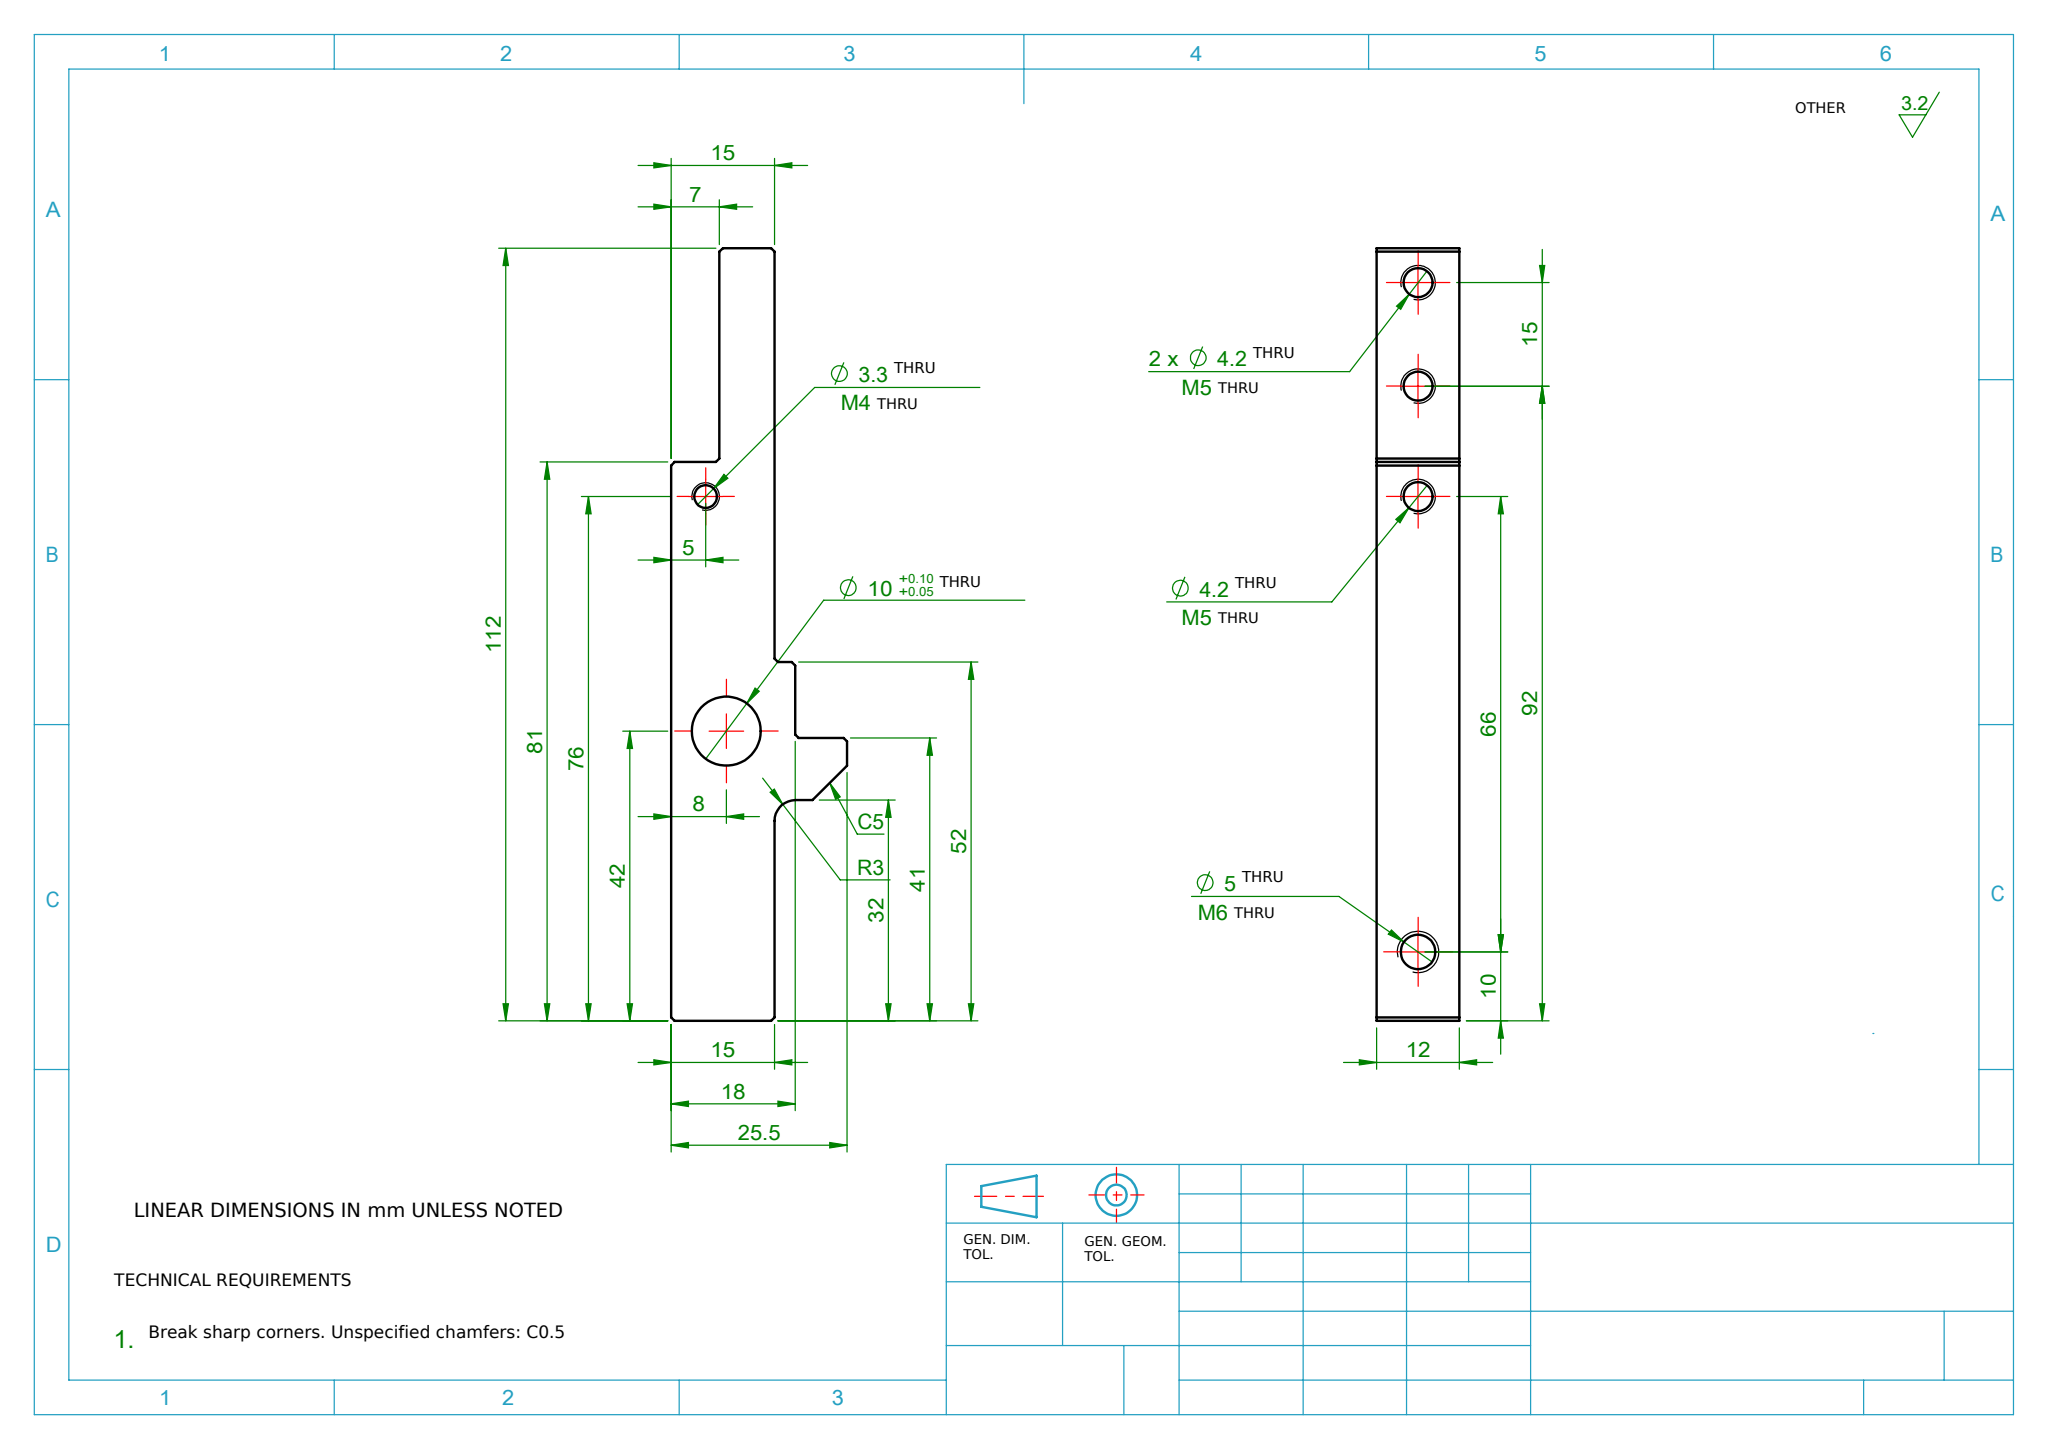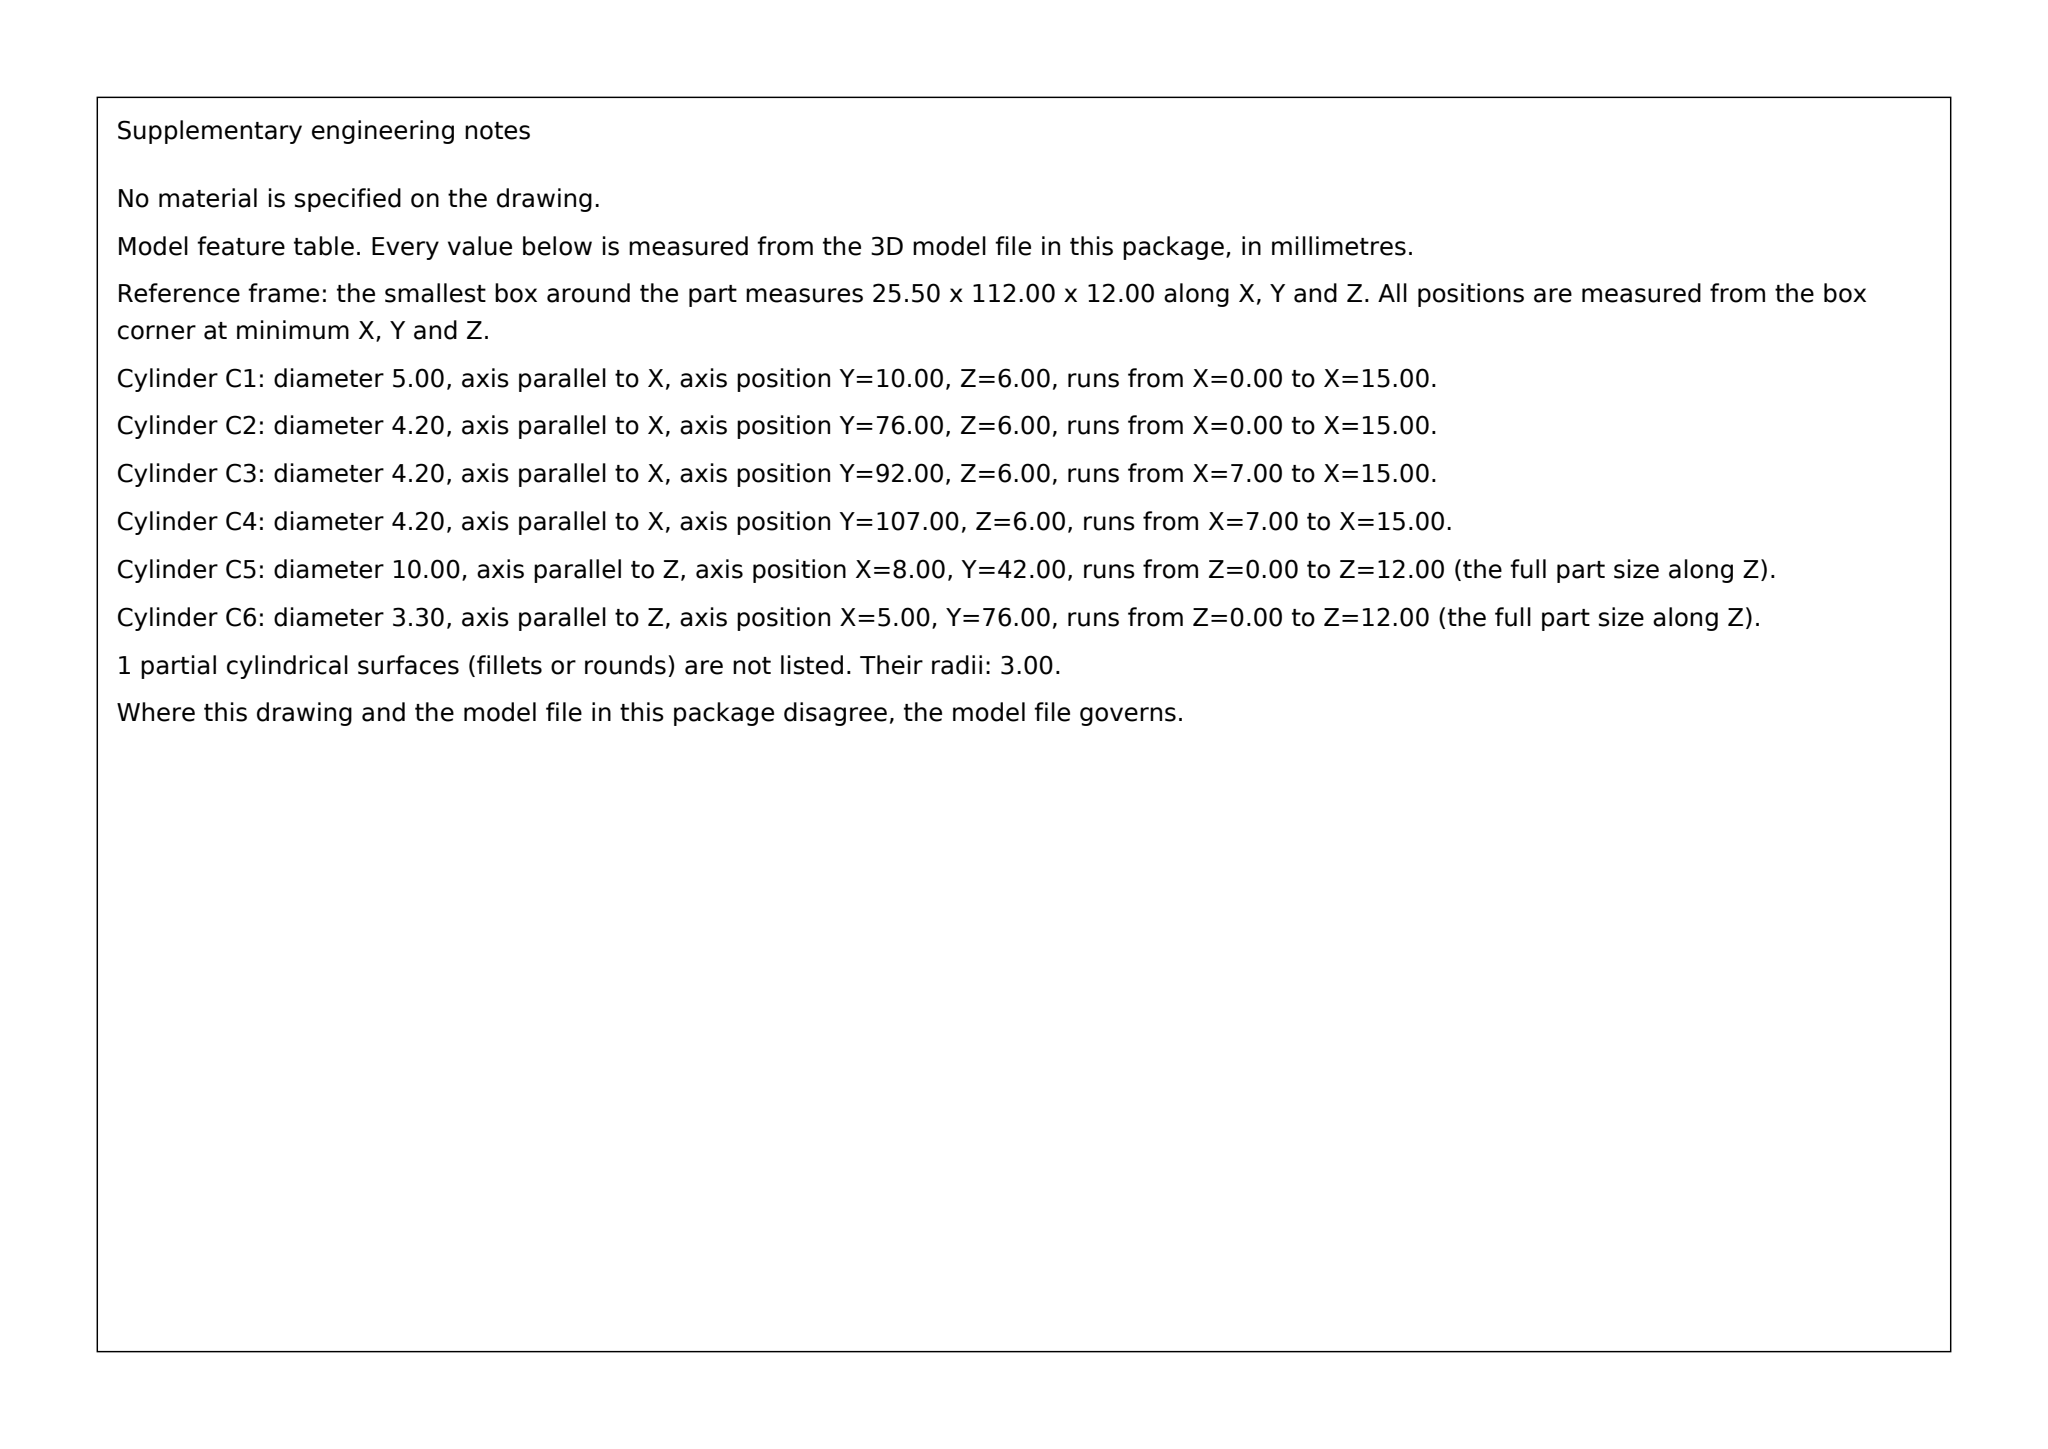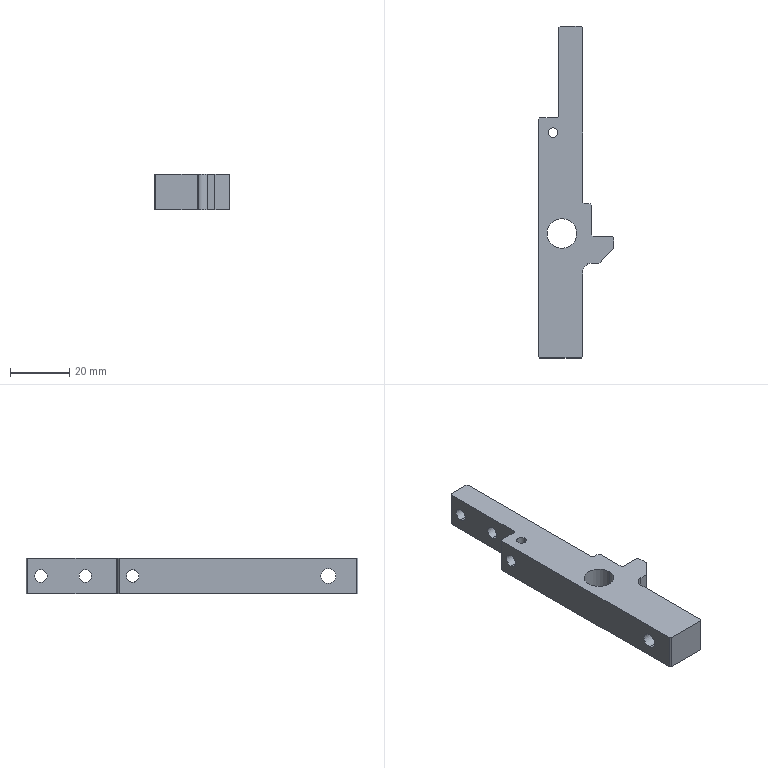Part | SolidWorks | mm | 1 solid | 40 faces | box 25.5 x 112 x 12 mm | volume 17217 mm3 | plane 25 | cylinder 15 | commonest cylinder face diameters 4.2 x6 3.3 x4 5 x2 10 x2 6 x1
build123d program:
from build123d import *

# Parameters (mm, degrees)
BOSS_EXTRUDE1_DEPTH       = 12
SIZE_MM_DOWEL_PIN_HOLE1_D = 10
M5_TAPPED_HOLE1_D         = 4.2
M4_TAPPED_HOLE1_D         = 3.3
M5_TAPPED_HOLE2_D         = 4.2
CHAMFER1_SIZE             = 0.5
M6_TAPPED_HOLE1_D         = 5
FILLET1_R                 = 3
CHAMFER2_SIZE             = 5


with BuildPart() as part:
    # Sketch1 → Boss-Extrude1 (new body)
    with BuildSketch(Plane.XY):
        Polygon((0, 0), (0, 81), (7, 81), (7, 112), (15, 112), (15, 52), (18, 52), (18, 41), (25.5, 41), (25.5, 32), (15, 32), (15, 0), align=None)
    extrude(amount=BOSS_EXTRUDE1_DEPTH)

    # Size mm Dowel Pin Hole1 (through all)
    with Locations(Plane.XY.offset(12)):
        with Locations((8, 42)):
            Hole(SIZE_MM_DOWEL_PIN_HOLE1_D / 2)

    # M5 Tapped Hole1 (through all)
    with Locations(Plane.ZY.offset(-7)):
        with Locations((6, 107), (6, 92)):
            Hole(M5_TAPPED_HOLE1_D / 2)

    # M4 Tapped Hole1 (through all)
    with Locations(Plane.XY.offset(12)):
        with Locations((5, 76)):
            Hole(M4_TAPPED_HOLE1_D / 2)

    # M5 Tapped Hole2 (through all)
    with Locations(Plane.ZY):
        with Locations((6, 76)):
            Hole(M5_TAPPED_HOLE2_D / 2)

    # Chamfer1
    chamfer1_edges = [part.edges().sort_by_distance(p)[0] for p in [
        (0, 0, 6),
        (0, 81, 6),
        (7, 81, 6),
        (7, 112, 6),
        (15, 112, 6),
        (15, 52, 6),
        (18, 52, 6),
        (18, 41, 6),
        (25.5, 41, 6),
        (15, 0, 6),
    ]]
    chamfer(chamfer1_edges, length=CHAMFER1_SIZE)

    # M6 Tapped Hole1 (through all)
    with Locations(Plane.ZY):
        with Locations((6, 10)):
            Hole(M6_TAPPED_HOLE1_D / 2)

    # Fillet1
    fillet1_edges = [part.edges().sort_by_distance(p)[0] for p in [
        (15, 32, 6),
    ]]
    fillet(fillet1_edges, radius=FILLET1_R)

    # Chamfer2
    chamfer2_edges = [part.edges().sort_by_distance(p)[0] for p in [
        (25.5, 32, 6),
    ]]
    chamfer(chamfer2_edges, length=CHAMFER2_SIZE)


solid = part.part